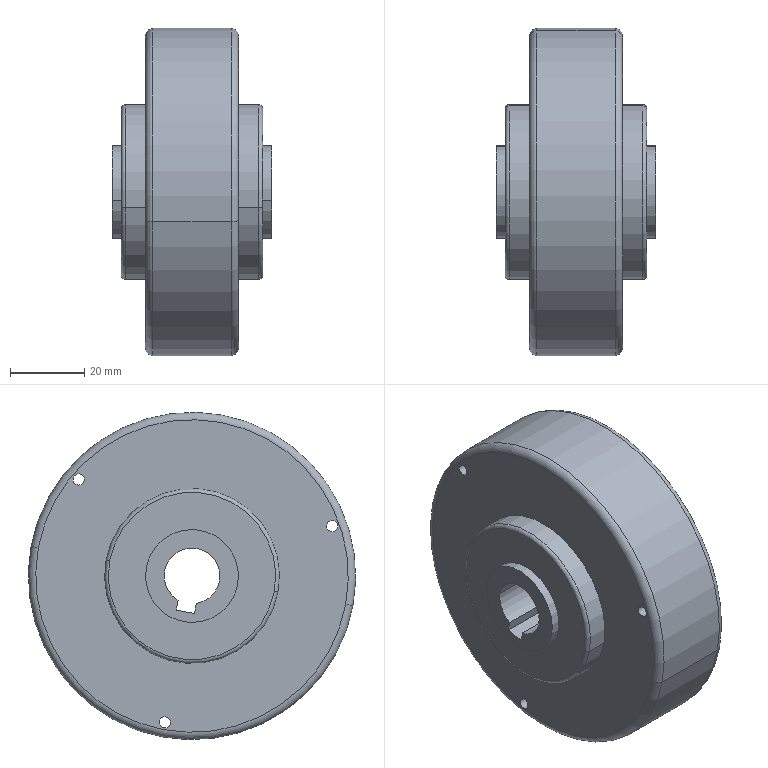Component | SolidWorks | PBT-003-1 | 1 solid | 36 faces | box 43 x 88 x 88 mm | volume 167875 mm3 | cylinder 19 | plane 9 | torus 8 | commonest cylinder face diameters 3 x6 25 x4 47 x4 15 x3 88 x2
build123d program:
from build123d import *

# Parameters (mm, degrees)
SKETCH1_R           = 44
BOSS_EXTRUDE1_DEPTH = 12.5
FILLET1_R           = 2
SKETCH2_R           = 23.5
BOSS_EXTRUDE2_DEPTH = 6.5
FILLET2_R           = 1
BOSS_EXTRUDE3_START = 6.5
SKETCH3_R           = 23.5
BOSS_EXTRUDE3_DEPTH = 6.5
FILLET3_R           = 1
CUT_EXTRUDE1_DEPTH  = 73.911
SKETCH5_R           = 1.5
CUT_EXTRUDE2_DEPTH  = 70.744
BOSS_EXTRUDE5_START = 2.5
SKETCH8_R           = 12.5
BOSS_EXTRUDE5_DEPTH = 2.5


with BuildPart() as part:
    # Sketch1 → Boss-Extrude1 (new, symmetric)
    with BuildSketch(Plane.XY):
        Circle(SKETCH1_R)
    extrude(amount=BOSS_EXTRUDE1_DEPTH, both=True)

    # Fillet1
    fillet1_edges = [part.edges().sort_by_distance(p)[0] for p in [
        (-44, 0, -12.5),
        (-44, 0, 12.5),
    ]]
    fillet(fillet1_edges, radius=FILLET1_R)

    # Sketch2 → Boss-Extrude2 (add)
    with BuildSketch(Plane.XY.offset(12.5)):
        with Locations(Location((0, 0, 0), (0, 0, 180))):
            Circle(SKETCH2_R)
    extrude(amount=BOSS_EXTRUDE2_DEPTH)

    # Fillet2
    fillet2_edges = [part.edges().sort_by_distance(p)[0] for p in [
        (23.5, 0, 19),
    ]]
    fillet(fillet2_edges, radius=FILLET2_R)

    # Sketch3 → Boss-Extrude3 (add)
    with BuildSketch(Plane(origin=(0, 0, -12.5), x_dir=(-1, 0, 0), z_dir=(0, 0, -1)).offset(BOSS_EXTRUDE3_START)):
        Circle(SKETCH3_R)
    extrude(amount=-BOSS_EXTRUDE3_DEPTH)

    # Fillet3
    fillet3_edges = [part.edges().sort_by_distance(p)[0] for p in [
        (23.5, 0, -19),
    ]]
    fillet(fillet3_edges, radius=FILLET3_R)

    # Sketch4 → Cut-Extrude1 (cut, through all)
    with BuildSketch(Plane.XY.offset(19)):
        with BuildLine():
            Line((2.5, 7.071), (2.5, 9.8))
            Line((2.5, 9.8), (-2.5, 9.8))
            Line((-2.5, 9.8), (-2.5, 7.071))
            ThreePointArc((-2.5, 7.071), (0, -7.5), (2.5, 7.071))
        make_face()
    extrude(amount=-CUT_EXTRUDE1_DEPTH, mode=Mode.SUBTRACT)

    # Sketch5 → Cut-Extrude2 (cut, through all)
    with BuildSketch(Plane.XY.offset(12.5)):
        with Locations((0, 40)):
            Circle(SKETCH5_R)
        with Locations((34.641, -20)):
            Circle(SKETCH5_R)
        with Locations((-34.641, -20)):
            Circle(SKETCH5_R)
    extrude(amount=-CUT_EXTRUDE2_DEPTH, mode=Mode.SUBTRACT)

    # Sketch8 → Boss-Extrude5 (add)
    with BuildSketch(Plane.XY.offset(19).offset(BOSS_EXTRUDE5_START)):
        Circle(SKETCH8_R)
        with BuildLine():
            Line((2.5, 7.071), (2.5, 9.8))
            Line((2.5, 9.8), (-2.5, 9.8))
            Line((-2.5, 9.8), (-2.5, 7.071))
            ThreePointArc((-2.5, 7.071), (0, -7.5), (2.5, 7.071))
        make_face(mode=Mode.SUBTRACT)
    boss_extrude5 = extrude(amount=-BOSS_EXTRUDE5_DEPTH)

    # Mirror1: Boss-Extrude5 across plane
    add(boss_extrude5.mirror(Plane.XY))


solid = part.part

# Placed as in the assembly
solid = solid.moved(Location((-51.784, -95.825, 207.018), (-79.544, 90, 0)))
STEP:
#1=CARTESIAN_POINT('',(-1.192,-3.289,8.24));
#2=VERTEX_POINT('',#1);
#3=CARTESIAN_POINT('',(-1.192,-4.257,8.061));
#4=VERTEX_POINT('',#3);
#5=CARTESIAN_POINT('',(-1.192,-3.773,8.15));
#6=DIRECTION('',(-1.,-0.,0.));
#7=DIRECTION('',(-0.,0.9834,0.1815));
#8=AXIS2_PLACEMENT_3D('',#5,#6,#7);
#9=CIRCLE('',#8,0.4921);
#10=EDGE_CURVE('',#2,#4,#9,.T.);
#11=ORIENTED_EDGE('',*,*,#10,.T.);
#12=CARTESIAN_POINT('',(-1.291,-4.257,8.061));
#13=VERTEX_POINT('',#12);
#14=CARTESIAN_POINT('',(-1.192,-4.257,8.061));
#15=DIRECTION('',(-1.,-0.,0.));
#16=VECTOR('',#15,39.37);
#17=LINE('',#14,#16);
#18=EDGE_CURVE('',#4,#13,#17,.T.);
#19=ORIENTED_EDGE('',*,*,#18,.T.);
#20=CARTESIAN_POINT('',(-1.291,-3.289,8.24));
#21=VERTEX_POINT('',#20);
#22=CARTESIAN_POINT('',(-1.291,-3.773,8.15));
#23=DIRECTION('',(1.,0.,-0.));
#24=DIRECTION('',(0.,-0.9834,-0.1815));
#25=AXIS2_PLACEMENT_3D('',#22,#23,#24);
#26=CIRCLE('',#25,0.4921);
#27=EDGE_CURVE('',#13,#21,#26,.T.);
#28=ORIENTED_EDGE('',*,*,#27,.T.);
#29=CARTESIAN_POINT('',(-1.192,-3.289,8.24));
#30=DIRECTION('',(-1.,-0.,0.));
#31=VECTOR('',#30,39.37);
#32=LINE('',#29,#31);
#33=EDGE_CURVE('',#2,#21,#32,.T.);
#34=ORIENTED_EDGE('',*,*,#33,.F.);
#35=EDGE_LOOP('',(#11,#19,#28,#34));
#36=FACE_OUTER_BOUND('',#35,.T.);
#37=CARTESIAN_POINT('',(-1.192,-3.773,8.15));
#38=DIRECTION('',(-1.,-0.,0.));
#39=DIRECTION('',(-0.,0.9834,0.1815));
#40=AXIS2_PLACEMENT_3D('',#37,#38,#39);
#41=CYLINDRICAL_SURFACE('',#40,0.4921);
#42=ADVANCED_FACE('',(#36),#41,.T.);
#43=CARTESIAN_POINT('',(-2.885,-3.289,8.24));
#44=VERTEX_POINT('',#43);
#45=CARTESIAN_POINT('',(-2.885,-4.257,8.061));
#46=VERTEX_POINT('',#45);
#47=CARTESIAN_POINT('',(-2.885,-3.773,8.15));
#48=DIRECTION('',(-1.,-0.,0.));
#49=DIRECTION('',(0.,0.9834,0.1815));
#50=AXIS2_PLACEMENT_3D('',#47,#48,#49);
#51=CIRCLE('',#50,0.4921);
#52=EDGE_CURVE('',#44,#46,#51,.T.);
#53=ORIENTED_EDGE('',*,*,#52,.F.);
#54=CARTESIAN_POINT('',(-2.787,-3.289,8.24));
#55=VERTEX_POINT('',#54);
#56=CARTESIAN_POINT('',(-2.885,-3.289,8.24));
#57=DIRECTION('',(1.,0.,-0.));
#58=VECTOR('',#57,39.37);
#59=LINE('',#56,#58);
#60=EDGE_CURVE('',#44,#55,#59,.T.);
#61=ORIENTED_EDGE('',*,*,#60,.T.);
#62=CARTESIAN_POINT('',(-2.787,-4.257,8.061));
#63=VERTEX_POINT('',#62);
#64=CARTESIAN_POINT('',(-2.787,-3.773,8.15));
#65=DIRECTION('',(-1.,-0.,0.));
#66=DIRECTION('',(0.,0.9834,0.1815));
#67=AXIS2_PLACEMENT_3D('',#64,#65,#66);
#68=CIRCLE('',#67,0.4921);
#69=EDGE_CURVE('',#55,#63,#68,.T.);
#70=ORIENTED_EDGE('',*,*,#69,.T.);
#71=CARTESIAN_POINT('',(-2.885,-4.257,8.061));
#72=DIRECTION('',(1.,0.,-0.));
#73=VECTOR('',#72,39.37);
#74=LINE('',#71,#73);
#75=EDGE_CURVE('',#46,#63,#74,.T.);
#76=ORIENTED_EDGE('',*,*,#75,.F.);
#77=EDGE_LOOP('',(#53,#61,#70,#76));
#78=FACE_OUTER_BOUND('',#77,.T.);
#79=CARTESIAN_POINT('',(-2.885,-3.773,8.15));
#80=DIRECTION('',(1.,0.,-0.));
#81=DIRECTION('',(0.,-0.9834,-0.1815));
#82=AXIS2_PLACEMENT_3D('',#79,#80,#81);
#83=CYLINDRICAL_SURFACE('',#82,0.4921);
#84=ADVANCED_FACE('',(#78),#83,.T.);
#85=CARTESIAN_POINT('',(-1.547,-5.315,8.666));
#86=VERTEX_POINT('',#85);
#87=CARTESIAN_POINT('',(-1.547,-5.199,8.688));
#88=VERTEX_POINT('',#87);
#89=CARTESIAN_POINT('',(-1.547,-5.257,8.677));
#90=DIRECTION('',(-1.,-0.,0.));
#91=DIRECTION('',(0.,0.9834,0.1815));
#92=AXIS2_PLACEMENT_3D('',#89,#90,#91);
#93=CIRCLE('',#92,0.05906);
#94=EDGE_CURVE('',#86,#88,#93,.T.);
#95=ORIENTED_EDGE('',*,*,#94,.F.);
#96=CARTESIAN_POINT('',(-2.531,-5.315,8.666));
#97=VERTEX_POINT('',#96);
#98=CARTESIAN_POINT('',(-1.291,-5.315,8.666));
#99=DIRECTION('',(-1.,-0.,0.));
#100=VECTOR('',#99,39.37);
#101=LINE('',#98,#100);
#102=EDGE_CURVE('',#86,#97,#101,.T.);
#103=ORIENTED_EDGE('',*,*,#102,.T.);
#104=CARTESIAN_POINT('',(-2.531,-5.199,8.688));
#105=VERTEX_POINT('',#104);
#106=CARTESIAN_POINT('',(-2.531,-5.257,8.677));
#107=DIRECTION('',(-1.,-0.,0.));
#108=DIRECTION('',(0.,0.9834,0.1815));
#109=AXIS2_PLACEMENT_3D('',#106,#107,#108);
#110=CIRCLE('',#109,0.05906);
#111=EDGE_CURVE('',#97,#105,#110,.T.);
#112=ORIENTED_EDGE('',*,*,#111,.T.);
#113=CARTESIAN_POINT('',(-1.291,-5.199,8.688));
#114=DIRECTION('',(-1.,-0.,0.));
#115=VECTOR('',#114,39.37);
#116=LINE('',#113,#115);
#117=EDGE_CURVE('',#88,#105,#116,.T.);
#118=ORIENTED_EDGE('',*,*,#117,.F.);
#119=EDGE_LOOP('',(#95,#103,#112,#118));
#120=FACE_OUTER_BOUND('',#119,.T.);
#121=CARTESIAN_POINT('',(-1.291,-5.257,8.677));
#122=DIRECTION('',(-1.,-0.,0.));
#123=DIRECTION('',(0.,0.9834,0.1815));
#124=AXIS2_PLACEMENT_3D('',#121,#122,#123);
#125=CYLINDRICAL_SURFACE('',#124,0.05906);
#126=ADVANCED_FACE('',(#120),#125,.F.);
#127=CARTESIAN_POINT('',(-1.547,-2.632,9.161));
#128=VERTEX_POINT('',#127);
#129=CARTESIAN_POINT('',(-1.547,-2.516,9.183));
#130=VERTEX_POINT('',#129);
#131=CARTESIAN_POINT('',(-1.547,-2.574,9.172));
#132=DIRECTION('',(-1.,-0.,0.));
#133=DIRECTION('',(0.,0.9834,0.1815));
#134=AXIS2_PLACEMENT_3D('',#131,#132,#133);
#135=CIRCLE('',#134,0.05906);
#136=EDGE_CURVE('',#128,#130,#135,.T.);
#137=ORIENTED_EDGE('',*,*,#136,.F.);
#138=CARTESIAN_POINT('',(-2.531,-2.632,9.161));
#139=VERTEX_POINT('',#138);
#140=CARTESIAN_POINT('',(-1.291,-2.632,9.161));
#141=DIRECTION('',(-1.,-0.,0.));
#142=VECTOR('',#141,39.37);
#143=LINE('',#140,#142);
#144=EDGE_CURVE('',#128,#139,#143,.T.);
#145=ORIENTED_EDGE('',*,*,#144,.T.);
#146=CARTESIAN_POINT('',(-2.531,-2.516,9.183));
#147=VERTEX_POINT('',#146);
#148=CARTESIAN_POINT('',(-2.531,-2.574,9.172));
#149=DIRECTION('',(-1.,-0.,0.));
#150=DIRECTION('',(0.,0.9834,0.1815));
#151=AXIS2_PLACEMENT_3D('',#148,#149,#150);
#152=CIRCLE('',#151,0.05906);
#153=EDGE_CURVE('',#139,#147,#152,.T.);
#154=ORIENTED_EDGE('',*,*,#153,.T.);
#155=CARTESIAN_POINT('',(-1.291,-2.516,9.183));
#156=DIRECTION('',(-1.,-0.,0.));
#157=VECTOR('',#156,39.37);
#158=LINE('',#155,#157);
#159=EDGE_CURVE('',#130,#147,#158,.T.);
#160=ORIENTED_EDGE('',*,*,#159,.F.);
#161=EDGE_LOOP('',(#137,#145,#154,#160));
#162=FACE_OUTER_BOUND('',#161,.T.);
#163=CARTESIAN_POINT('',(-1.291,-2.574,9.172));
#164=DIRECTION('',(-1.,-0.,0.));
#165=DIRECTION('',(0.,0.9834,0.1815));
#166=AXIS2_PLACEMENT_3D('',#163,#164,#165);
#167=CYLINDRICAL_SURFACE('',#166,0.05906);
#168=ADVANCED_FACE('',(#162),#167,.F.);
#169=CARTESIAN_POINT('',(-1.547,-3.545,6.591));
#170=VERTEX_POINT('',#169);
#171=CARTESIAN_POINT('',(-1.547,-3.429,6.612));
#172=VERTEX_POINT('',#171);
#173=CARTESIAN_POINT('',(-1.547,-3.487,6.602));
#174=DIRECTION('',(-1.,-0.,0.));
#175=DIRECTION('',(0.,0.9834,0.1815));
#176=AXIS2_PLACEMENT_3D('',#173,#174,#175);
#177=CIRCLE('',#176,0.05906);
#178=EDGE_CURVE('',#170,#172,#177,.T.);
#179=ORIENTED_EDGE('',*,*,#178,.F.);
#180=CARTESIAN_POINT('',(-2.531,-3.545,6.591));
#181=VERTEX_POINT('',#180);
#182=CARTESIAN_POINT('',(-1.291,-3.545,6.591));
#183=DIRECTION('',(-1.,-0.,0.));
#184=VECTOR('',#183,39.37);
#185=LINE('',#182,#184);
#186=EDGE_CURVE('',#170,#181,#185,.T.);
#187=ORIENTED_EDGE('',*,*,#186,.T.);
#188=CARTESIAN_POINT('',(-2.531,-3.429,6.612));
#189=VERTEX_POINT('',#188);
#190=CARTESIAN_POINT('',(-2.531,-3.487,6.602));
#191=DIRECTION('',(-1.,-0.,0.));
#192=DIRECTION('',(0.,0.9834,0.1815));
#193=AXIS2_PLACEMENT_3D('',#190,#191,#192);
#194=CIRCLE('',#193,0.05906);
#195=EDGE_CURVE('',#181,#189,#194,.T.);
#196=ORIENTED_EDGE('',*,*,#195,.T.);
#197=CARTESIAN_POINT('',(-1.291,-3.429,6.612));
#198=DIRECTION('',(-1.,-0.,0.));
#199=VECTOR('',#198,39.37);
#200=LINE('',#197,#199);
#201=EDGE_CURVE('',#172,#189,#200,.T.);
#202=ORIENTED_EDGE('',*,*,#201,.F.);
#203=EDGE_LOOP('',(#179,#187,#196,#202));
#204=FACE_OUTER_BOUND('',#203,.T.);
#205=CARTESIAN_POINT('',(-1.291,-3.487,6.602));
#206=DIRECTION('',(-1.,-0.,0.));
#207=DIRECTION('',(0.,0.9834,0.1815));
#208=AXIS2_PLACEMENT_3D('',#205,#206,#207);
#209=CYLINDRICAL_SURFACE('',#208,0.05906);
#210=ADVANCED_FACE('',(#204),#209,.F.);
#211=CARTESIAN_POINT('',(-1.192,-4.063,8.097));
#212=VERTEX_POINT('',#211);
#213=CARTESIAN_POINT('',(-1.192,-3.482,8.204));
#214=VERTEX_POINT('',#213);
#215=CARTESIAN_POINT('',(-1.192,-3.773,8.15));
#216=DIRECTION('',(-1.,-0.,0.));
#217=DIRECTION('',(-0.,0.9834,0.1815));
#218=AXIS2_PLACEMENT_3D('',#215,#216,#217);
#219=CIRCLE('',#218,0.2953);
#220=EDGE_CURVE('',#212,#214,#219,.T.);
#221=ORIENTED_EDGE('',*,*,#220,.F.);
#222=CARTESIAN_POINT('',(-2.885,-4.063,8.097));
#223=VERTEX_POINT('',#222);
#224=CARTESIAN_POINT('',(-1.291,-4.063,8.097));
#225=DIRECTION('',(-1.,-0.,0.));
#226=VECTOR('',#225,39.37);
#227=LINE('',#224,#226);
#228=EDGE_CURVE('',#212,#223,#227,.T.);
#229=ORIENTED_EDGE('',*,*,#228,.T.);
#230=CARTESIAN_POINT('',(-2.885,-3.482,8.204));
#231=VERTEX_POINT('',#230);
#232=CARTESIAN_POINT('',(-2.885,-3.773,8.15));
#233=DIRECTION('',(-1.,-0.,0.));
#234=DIRECTION('',(0.,0.9834,0.1815));
#235=AXIS2_PLACEMENT_3D('',#232,#233,#234);
#236=CIRCLE('',#235,0.2953);
#237=EDGE_CURVE('',#223,#231,#236,.T.);
#238=ORIENTED_EDGE('',*,*,#237,.T.);
#239=CARTESIAN_POINT('',(-1.291,-3.482,8.204));
#240=DIRECTION('',(-1.,-0.,0.));
#241=VECTOR('',#240,39.37);
#242=LINE('',#239,#241);
#243=EDGE_CURVE('',#214,#231,#242,.T.);
#244=ORIENTED_EDGE('',*,*,#243,.F.);
#245=EDGE_LOOP('',(#221,#229,#238,#244));
#246=FACE_OUTER_BOUND('',#245,.T.);
#247=CARTESIAN_POINT('',(-1.291,-3.773,8.15));
#248=DIRECTION('',(-1.,-0.,0.));
#249=DIRECTION('',(0.,0.9834,0.1815));
#250=AXIS2_PLACEMENT_3D('',#247,#248,#249);
#251=CYLINDRICAL_SURFACE('',#250,0.2953);
#252=ADVANCED_FACE('',(#246),#251,.F.);
#253=CARTESIAN_POINT('',(-1.192,-3.625,7.894));
#254=VERTEX_POINT('',#253);
#255=CARTESIAN_POINT('',(-1.192,-3.773,8.15));
#256=DIRECTION('',(-1.,-0.,0.));
#257=DIRECTION('',(-0.,0.9834,0.1815));
#258=AXIS2_PLACEMENT_3D('',#255,#256,#257);
#259=CIRCLE('',#258,0.2953);
#260=EDGE_CURVE('',#214,#254,#259,.T.);
#261=ORIENTED_EDGE('',*,*,#260,.F.);
#262=ORIENTED_EDGE('',*,*,#243,.T.);
#263=CARTESIAN_POINT('',(-2.885,-3.625,7.894));
#264=VERTEX_POINT('',#263);
#265=CARTESIAN_POINT('',(-2.885,-3.773,8.15));
#266=DIRECTION('',(-1.,-0.,0.));
#267=DIRECTION('',(0.,0.9834,0.1815));
#268=AXIS2_PLACEMENT_3D('',#265,#266,#267);
#269=CIRCLE('',#268,0.2953);
#270=EDGE_CURVE('',#231,#264,#269,.T.);
#271=ORIENTED_EDGE('',*,*,#270,.T.);
#272=CARTESIAN_POINT('',(-1.291,-3.625,7.894));
#273=DIRECTION('',(-1.,-0.,0.));
#274=VECTOR('',#273,39.37);
#275=LINE('',#272,#274);
#276=EDGE_CURVE('',#254,#264,#275,.T.);
#277=ORIENTED_EDGE('',*,*,#276,.F.);
#278=EDGE_LOOP('',(#261,#262,#271,#277));
#279=FACE_OUTER_BOUND('',#278,.T.);
#280=CARTESIAN_POINT('',(-1.291,-3.773,8.15));
#281=DIRECTION('',(-1.,-0.,0.));
#282=DIRECTION('',(0.,0.9834,0.1815));
#283=AXIS2_PLACEMENT_3D('',#280,#281,#282);
#284=CYLINDRICAL_SURFACE('',#283,0.2953);
#285=ADVANCED_FACE('',(#279),#284,.F.);
#286=CARTESIAN_POINT('',(-1.33,-2.863,8.318));
#287=VERTEX_POINT('',#286);
#288=CARTESIAN_POINT('',(-1.33,-4.682,7.982));
#289=VERTEX_POINT('',#288);
#290=CARTESIAN_POINT('',(-1.33,-3.773,8.15));
#291=DIRECTION('',(-1.,-0.,0.));
#292=DIRECTION('',(0.,-0.9834,-0.1815));
#293=AXIS2_PLACEMENT_3D('',#290,#291,#292);
#294=CIRCLE('',#293,0.9252);
#295=EDGE_CURVE('',#287,#289,#294,.T.);
#296=ORIENTED_EDGE('',*,*,#295,.F.);
#297=CARTESIAN_POINT('',(-1.291,-2.902,8.311));
#298=VERTEX_POINT('',#297);
#299=CARTESIAN_POINT('',(-1.33,-2.902,8.311));
#300=DIRECTION('',(-0.,0.1815,-0.9834));
#301=DIRECTION('',(0.,0.9834,0.1815));
#302=AXIS2_PLACEMENT_3D('',#299,#300,#301);
#303=CIRCLE('',#302,0.03937);
#304=EDGE_CURVE('',#287,#298,#303,.T.);
#305=ORIENTED_EDGE('',*,*,#304,.T.);
#306=CARTESIAN_POINT('',(-1.291,-4.644,7.99));
#307=VERTEX_POINT('',#306);
#308=CARTESIAN_POINT('',(-1.291,-3.773,8.15));
#309=DIRECTION('',(1.,0.,-0.));
#310=DIRECTION('',(0.,-0.9834,-0.1815));
#311=AXIS2_PLACEMENT_3D('',#308,#309,#310);
#312=CIRCLE('',#311,0.8858);
#313=EDGE_CURVE('',#307,#298,#312,.T.);
#314=ORIENTED_EDGE('',*,*,#313,.F.);
#315=CARTESIAN_POINT('',(-1.33,-4.644,7.99));
#316=DIRECTION('',(0.,-0.1815,0.9834));
#317=DIRECTION('',(0.,-0.9834,-0.1815));
#318=AXIS2_PLACEMENT_3D('',#315,#316,#317);
#319=CIRCLE('',#318,0.03937);
#320=EDGE_CURVE('',#289,#307,#319,.T.);
#321=ORIENTED_EDGE('',*,*,#320,.F.);
#322=EDGE_LOOP('',(#296,#305,#314,#321));
#323=FACE_OUTER_BOUND('',#322,.T.);
#324=CARTESIAN_POINT('',(-1.33,-3.773,8.15));
#325=DIRECTION('',(1.,0.,-0.));
#326=DIRECTION('',(0.,-0.9834,-0.1815));
#327=AXIS2_PLACEMENT_3D('',#324,#325,#326);
#328=TOROIDAL_SURFACE('',#327,0.8858,0.03937);
#329=ADVANCED_FACE('',(#323),#328,.T.);
#330=ORIENTED_EDGE('',*,*,#295,.T.);
#331=CARTESIAN_POINT('',(-1.547,-4.682,7.982));
#332=VERTEX_POINT('',#331);
#333=CARTESIAN_POINT('',(-1.291,-4.682,7.982));
#334=DIRECTION('',(-1.,-0.,0.));
#335=VECTOR('',#334,39.37);
#336=LINE('',#333,#335);
#337=EDGE_CURVE('',#289,#332,#336,.T.);
#338=ORIENTED_EDGE('',*,*,#337,.T.);
#339=CARTESIAN_POINT('',(-1.547,-2.863,8.318));
#340=VERTEX_POINT('',#339);
#341=CARTESIAN_POINT('',(-1.547,-3.773,8.15));
#342=DIRECTION('',(1.,0.,-0.));
#343=DIRECTION('',(-0.,0.9834,0.1815));
#344=AXIS2_PLACEMENT_3D('',#341,#342,#343);
#345=CIRCLE('',#344,0.9252);
#346=EDGE_CURVE('',#332,#340,#345,.T.);
#347=ORIENTED_EDGE('',*,*,#346,.T.);
#348=CARTESIAN_POINT('',(-1.291,-2.863,8.318));
#349=DIRECTION('',(-1.,-0.,0.));
#350=VECTOR('',#349,39.37);
#351=LINE('',#348,#350);
#352=EDGE_CURVE('',#287,#340,#351,.T.);
#353=ORIENTED_EDGE('',*,*,#352,.F.);
#354=EDGE_LOOP('',(#330,#338,#347,#353));
#355=FACE_OUTER_BOUND('',#354,.T.);
#356=CARTESIAN_POINT('',(-1.291,-3.773,8.15));
#357=DIRECTION('',(-1.,-0.,0.));
#358=DIRECTION('',(-0.,0.9834,0.1815));
#359=AXIS2_PLACEMENT_3D('',#356,#357,#358);
#360=CYLINDRICAL_SURFACE('',#359,0.9252);
#361=ADVANCED_FACE('',(#355),#360,.T.);
#362=CARTESIAN_POINT('',(-2.747,-4.682,7.982));
#363=VERTEX_POINT('',#362);
#364=CARTESIAN_POINT('',(-2.747,-2.863,8.318));
#365=VERTEX_POINT('',#364);
#366=CARTESIAN_POINT('',(-2.747,-3.773,8.15));
#367=DIRECTION('',(1.,0.,-0.));
#368=DIRECTION('',(0.,0.9834,0.1815));
#369=AXIS2_PLACEMENT_3D('',#366,#367,#368);
#370=CIRCLE('',#369,0.9252);
#371=EDGE_CURVE('',#363,#365,#370,.T.);
#372=ORIENTED_EDGE('',*,*,#371,.F.);
#373=CARTESIAN_POINT('',(-2.787,-4.644,7.99));
#374=VERTEX_POINT('',#373);
#375=CARTESIAN_POINT('',(-2.747,-4.644,7.99));
#376=DIRECTION('',(-0.,0.1815,-0.9834));
#377=DIRECTION('',(0.,0.9834,0.1815));
#378=AXIS2_PLACEMENT_3D('',#375,#376,#377);
#379=CIRCLE('',#378,0.03937);
#380=EDGE_CURVE('',#363,#374,#379,.T.);
#381=ORIENTED_EDGE('',*,*,#380,.T.);
#382=CARTESIAN_POINT('',(-2.787,-2.902,8.311));
#383=VERTEX_POINT('',#382);
#384=CARTESIAN_POINT('',(-2.787,-3.773,8.15));
#385=DIRECTION('',(-1.,-0.,0.));
#386=DIRECTION('',(0.,0.9834,0.1815));
#387=AXIS2_PLACEMENT_3D('',#384,#385,#386);
#388=CIRCLE('',#387,0.8858);
#389=EDGE_CURVE('',#383,#374,#388,.T.);
#390=ORIENTED_EDGE('',*,*,#389,.F.);
#391=CARTESIAN_POINT('',(-2.747,-2.902,8.311));
#392=DIRECTION('',(0.,-0.1815,0.9834));
#393=DIRECTION('',(0.,-0.9834,-0.1815));
#394=AXIS2_PLACEMENT_3D('',#391,#392,#393);
#395=CIRCLE('',#394,0.03937);
#396=EDGE_CURVE('',#365,#383,#395,.T.);
#397=ORIENTED_EDGE('',*,*,#396,.F.);
#398=EDGE_LOOP('',(#372,#381,#390,#397));
#399=FACE_OUTER_BOUND('',#398,.T.);
#400=CARTESIAN_POINT('',(-2.747,-3.773,8.15));
#401=DIRECTION('',(-1.,-0.,0.));
#402=DIRECTION('',(-0.,0.9834,0.1815));
#403=AXIS2_PLACEMENT_3D('',#400,#401,#402);
#404=TOROIDAL_SURFACE('',#403,0.8858,0.03937);
#405=ADVANCED_FACE('',(#399),#404,.T.);
#406=ORIENTED_EDGE('',*,*,#371,.T.);
#407=CARTESIAN_POINT('',(-2.531,-2.863,8.318));
#408=VERTEX_POINT('',#407);
#409=CARTESIAN_POINT('',(-2.787,-2.863,8.318));
#410=DIRECTION('',(1.,0.,-0.));
#411=VECTOR('',#410,39.37);
#412=LINE('',#409,#411);
#413=EDGE_CURVE('',#365,#408,#412,.T.);
#414=ORIENTED_EDGE('',*,*,#413,.T.);
#415=CARTESIAN_POINT('',(-2.531,-4.682,7.982));
#416=VERTEX_POINT('',#415);
#417=CARTESIAN_POINT('',(-2.531,-3.773,8.15));
#418=DIRECTION('',(-1.,-0.,0.));
#419=DIRECTION('',(0.,0.9834,0.1815));
#420=AXIS2_PLACEMENT_3D('',#417,#418,#419);
#421=CIRCLE('',#420,0.9252);
#422=EDGE_CURVE('',#408,#416,#421,.T.);
#423=ORIENTED_EDGE('',*,*,#422,.T.);
#424=CARTESIAN_POINT('',(-2.787,-4.682,7.982));
#425=DIRECTION('',(1.,0.,-0.));
#426=VECTOR('',#425,39.37);
#427=LINE('',#424,#426);
#428=EDGE_CURVE('',#363,#416,#427,.T.);
#429=ORIENTED_EDGE('',*,*,#428,.F.);
#430=EDGE_LOOP('',(#406,#414,#423,#429));
#431=FACE_OUTER_BOUND('',#430,.T.);
#432=CARTESIAN_POINT('',(-2.787,-3.773,8.15));
#433=DIRECTION('',(1.,0.,-0.));
#434=DIRECTION('',(0.,-0.9834,-0.1815));
#435=AXIS2_PLACEMENT_3D('',#432,#433,#434);
#436=CYLINDRICAL_SURFACE('',#435,0.9252);
#437=ADVANCED_FACE('',(#431),#436,.T.);
#438=CARTESIAN_POINT('',(-2.452,-5.476,7.836));
#439=VERTEX_POINT('',#438);
#440=CARTESIAN_POINT('',(-2.452,-2.069,8.465));
#441=VERTEX_POINT('',#440);
#442=CARTESIAN_POINT('',(-2.452,-3.773,8.15));
#443=DIRECTION('',(1.,0.,-0.));
#444=DIRECTION('',(-0.,0.9834,0.1815));
#445=AXIS2_PLACEMENT_3D('',#442,#443,#444);
#446=CIRCLE('',#445,1.732);
#447=EDGE_CURVE('',#439,#441,#446,.T.);
#448=ORIENTED_EDGE('',*,*,#447,.F.);
#449=CARTESIAN_POINT('',(-2.531,-5.399,7.85));
#450=VERTEX_POINT('',#449);
#451=CARTESIAN_POINT('',(-2.452,-5.399,7.85));
#452=DIRECTION('',(-0.,0.1815,-0.9834));
#453=DIRECTION('',(0.,0.9834,0.1815));
#454=AXIS2_PLACEMENT_3D('',#451,#452,#453);
#455=CIRCLE('',#454,0.07874);
#456=EDGE_CURVE('',#439,#450,#455,.T.);
#457=ORIENTED_EDGE('',*,*,#456,.T.);
#458=CARTESIAN_POINT('',(-2.531,-2.147,8.45));
#459=VERTEX_POINT('',#458);
#460=CARTESIAN_POINT('',(-2.531,-3.773,8.15));
#461=DIRECTION('',(-1.,-0.,0.));
#462=DIRECTION('',(-0.,0.9834,0.1815));
#463=AXIS2_PLACEMENT_3D('',#460,#461,#462);
#464=CIRCLE('',#463,1.654);
#465=EDGE_CURVE('',#459,#450,#464,.T.);
#466=ORIENTED_EDGE('',*,*,#465,.F.);
#467=CARTESIAN_POINT('',(-2.452,-2.147,8.45));
#468=DIRECTION('',(0.,-0.1815,0.9834));
#469=DIRECTION('',(0.,-0.9834,-0.1815));
#470=AXIS2_PLACEMENT_3D('',#467,#468,#469);
#471=CIRCLE('',#470,0.07874);
#472=EDGE_CURVE('',#441,#459,#471,.T.);
#473=ORIENTED_EDGE('',*,*,#472,.F.);
#474=EDGE_LOOP('',(#448,#457,#466,#473));
#475=FACE_OUTER_BOUND('',#474,.T.);
#476=CARTESIAN_POINT('',(-2.452,-3.773,8.15));
#477=DIRECTION('',(-1.,-0.,0.));
#478=DIRECTION('',(-0.,0.9834,0.1815));
#479=AXIS2_PLACEMENT_3D('',#476,#477,#478);
#480=TOROIDAL_SURFACE('',#479,1.654,0.07874);
#481=ADVANCED_FACE('',(#475),#480,.T.);
#482=CARTESIAN_POINT('',(-1.547,-5.399,7.85));
#483=VERTEX_POINT('',#482);
#484=CARTESIAN_POINT('',(-1.547,-2.147,8.45));
#485=VERTEX_POINT('',#484);
#486=CARTESIAN_POINT('',(-1.547,-3.773,8.15));
#487=DIRECTION('',(1.,0.,-0.));
#488=DIRECTION('',(-0.,0.9834,0.1815));
#489=AXIS2_PLACEMENT_3D('',#486,#487,#488);
#490=CIRCLE('',#489,1.654);
#491=EDGE_CURVE('',#483,#485,#490,.T.);
#492=ORIENTED_EDGE('',*,*,#491,.F.);
#493=CARTESIAN_POINT('',(-1.625,-5.476,7.836));
#494=VERTEX_POINT('',#493);
#495=CARTESIAN_POINT('',(-1.625,-5.399,7.85));
#496=DIRECTION('',(-0.,0.1815,-0.9834));
#497=DIRECTION('',(0.,0.9834,0.1815));
#498=AXIS2_PLACEMENT_3D('',#495,#496,#497);
#499=CIRCLE('',#498,0.07874);
#500=EDGE_CURVE('',#483,#494,#499,.T.);
#501=ORIENTED_EDGE('',*,*,#500,.T.);
#502=CARTESIAN_POINT('',(-1.625,-2.069,8.465));
#503=VERTEX_POINT('',#502);
#504=CARTESIAN_POINT('',(-1.625,-3.773,8.15));
#505=DIRECTION('',(-1.,-0.,0.));
#506=DIRECTION('',(-0.,0.9834,0.1815));
#507=AXIS2_PLACEMENT_3D('',#504,#505,#506);
#508=CIRCLE('',#507,1.732);
#509=EDGE_CURVE('',#503,#494,#508,.T.);
#510=ORIENTED_EDGE('',*,*,#509,.F.);
#511=CARTESIAN_POINT('',(-1.625,-2.147,8.45));
#512=DIRECTION('',(0.,-0.1815,0.9834));
#513=DIRECTION('',(0.,-0.9834,-0.1815));
#514=AXIS2_PLACEMENT_3D('',#511,#512,#513);
#515=CIRCLE('',#514,0.07874);
#516=EDGE_CURVE('',#485,#503,#515,.T.);
#517=ORIENTED_EDGE('',*,*,#516,.F.);
#518=EDGE_LOOP('',(#492,#501,#510,#517));
#519=FACE_OUTER_BOUND('',#518,.T.);
#520=CARTESIAN_POINT('',(-1.625,-3.773,8.15));
#521=DIRECTION('',(-1.,-0.,0.));
#522=DIRECTION('',(-0.,0.9834,0.1815));
#523=AXIS2_PLACEMENT_3D('',#520,#521,#522);
#524=TOROIDAL_SURFACE('',#523,1.654,0.07874);
#525=ADVANCED_FACE('',(#519),#524,.T.);
#526=ORIENTED_EDGE('',*,*,#447,.T.);
#527=CARTESIAN_POINT('',(-2.531,-2.069,8.465));
#528=DIRECTION('',(1.,0.,-0.));
#529=VECTOR('',#528,39.37);
#530=LINE('',#527,#529);
#531=EDGE_CURVE('',#441,#503,#530,.T.);
#532=ORIENTED_EDGE('',*,*,#531,.T.);
#533=ORIENTED_EDGE('',*,*,#509,.T.);
#534=CARTESIAN_POINT('',(-2.531,-5.476,7.836));
#535=DIRECTION('',(1.,0.,-0.));
#536=VECTOR('',#535,39.37);
#537=LINE('',#534,#536);
#538=EDGE_CURVE('',#439,#494,#537,.T.);
#539=ORIENTED_EDGE('',*,*,#538,.F.);
#540=EDGE_LOOP('',(#526,#532,#533,#539));
#541=FACE_OUTER_BOUND('',#540,.T.);
#542=CARTESIAN_POINT('',(-2.531,-3.773,8.15));
#543=DIRECTION('',(1.,0.,-0.));
#544=DIRECTION('',(0.,-0.9834,-0.1815));
#545=AXIS2_PLACEMENT_3D('',#542,#543,#544);
#546=CYLINDRICAL_SURFACE('',#545,1.732);
#547=ADVANCED_FACE('',(#541),#546,.T.);
#548=ORIENTED_EDGE('',*,*,#389,.T.);
#549=CARTESIAN_POINT('',(-2.787,-3.773,8.15));
#550=DIRECTION('',(-1.,-0.,0.));
#551=DIRECTION('',(0.,0.9834,0.1815));
#552=AXIS2_PLACEMENT_3D('',#549,#550,#551);
#553=CIRCLE('',#552,0.8858);
#554=EDGE_CURVE('',#374,#383,#553,.T.);
#555=ORIENTED_EDGE('',*,*,#554,.T.);
#556=EDGE_LOOP('',(#548,#555));
#557=FACE_OUTER_BOUND('',#556,.T.);
#558=CARTESIAN_POINT('',(-2.787,-3.773,8.15));
#559=DIRECTION('',(-1.,-0.,0.));
#560=DIRECTION('',(0.,0.9834,0.1815));
#561=AXIS2_PLACEMENT_3D('',#558,#559,#560);
#562=CIRCLE('',#561,0.4921);
#563=EDGE_CURVE('',#63,#55,#562,.T.);
#564=ORIENTED_EDGE('',*,*,#563,.F.);
#565=ORIENTED_EDGE('',*,*,#69,.F.);
#566=EDGE_LOOP('',(#564,#565));
#567=FACE_BOUND('',#566,.T.);
#568=CARTESIAN_POINT('',(-2.787,-3.773,8.15));
#569=DIRECTION('',(-1.,-0.,0.));
#570=DIRECTION('',(-0.,0.9834,0.1815));
#571=AXIS2_PLACEMENT_3D('',#568,#569,#570);
#572=PLANE('',#571);
#573=ADVANCED_FACE('',(#557,#567),#572,.T.);
#574=CARTESIAN_POINT('',(-1.547,-5.257,8.677));
#575=DIRECTION('',(-1.,-0.,0.));
#576=DIRECTION('',(0.,0.9834,0.1815));
#577=AXIS2_PLACEMENT_3D('',#574,#575,#576);
#578=CIRCLE('',#577,0.05906);
#579=EDGE_CURVE('',#88,#86,#578,.T.);
#580=ORIENTED_EDGE('',*,*,#579,.T.);
#581=ORIENTED_EDGE('',*,*,#94,.T.);
#582=EDGE_LOOP('',(#580,#581));
#583=FACE_BOUND('',#582,.T.);
#584=CARTESIAN_POINT('',(-1.547,-2.574,9.172));
#585=DIRECTION('',(-1.,-0.,0.));
#586=DIRECTION('',(0.,0.9834,0.1815));
#587=AXIS2_PLACEMENT_3D('',#584,#585,#586);
#588=CIRCLE('',#587,0.05906);
#589=EDGE_CURVE('',#130,#128,#588,.T.);
#590=ORIENTED_EDGE('',*,*,#589,.T.);
#591=ORIENTED_EDGE('',*,*,#136,.T.);
#592=EDGE_LOOP('',(#590,#591));
#593=FACE_BOUND('',#592,.T.);
#594=CARTESIAN_POINT('',(-1.547,-3.487,6.602));
#595=DIRECTION('',(-1.,-0.,0.));
#596=DIRECTION('',(0.,0.9834,0.1815));
#597=AXIS2_PLACEMENT_3D('',#594,#595,#596);
#598=CIRCLE('',#597,0.05906);
#599=EDGE_CURVE('',#172,#170,#598,.T.);
#600=ORIENTED_EDGE('',*,*,#599,.T.);
#601=ORIENTED_EDGE('',*,*,#178,.T.);
#602=EDGE_LOOP('',(#600,#601));
#603=FACE_BOUND('',#602,.T.);
#604=CARTESIAN_POINT('',(-1.547,-3.773,8.15));
#605=DIRECTION('',(1.,0.,-0.));
#606=DIRECTION('',(-0.,0.9834,0.1815));
#607=AXIS2_PLACEMENT_3D('',#604,#605,#606);
#608=CIRCLE('',#607,1.654);
#609=EDGE_CURVE('',#485,#483,#608,.T.);
#610=ORIENTED_EDGE('',*,*,#609,.T.);
#611=ORIENTED_EDGE('',*,*,#491,.T.);
#612=EDGE_LOOP('',(#610,#611));
#613=FACE_OUTER_BOUND('',#612,.T.);
#614=CARTESIAN_POINT('',(-1.547,-3.773,8.15));
#615=DIRECTION('',(1.,0.,-0.));
#616=DIRECTION('',(-0.,0.9834,0.1815));
#617=AXIS2_PLACEMENT_3D('',#614,#615,#616);
#618=CIRCLE('',#617,0.9252);
#619=EDGE_CURVE('',#340,#332,#618,.T.);
#620=ORIENTED_EDGE('',*,*,#619,.F.);
#621=ORIENTED_EDGE('',*,*,#346,.F.);
#622=EDGE_LOOP('',(#620,#621));
#623=FACE_BOUND('',#622,.T.);
#624=CARTESIAN_POINT('',(-1.547,-3.773,8.15));
#625=DIRECTION('',(-1.,-0.,0.));
#626=DIRECTION('',(-0.,0.9834,0.1815));
#627=AXIS2_PLACEMENT_3D('',#624,#625,#626);
#628=PLANE('',#627);
#629=ADVANCED_FACE('',(#583,#593,#603,#613,#623),#628,.F.);
#630=CARTESIAN_POINT('',(-2.531,-5.257,8.677));
#631=DIRECTION('',(-1.,-0.,0.));
#632=DIRECTION('',(0.,0.9834,0.1815));
#633=AXIS2_PLACEMENT_3D('',#630,#631,#632);
#634=CIRCLE('',#633,0.05906);
#635=EDGE_CURVE('',#105,#97,#634,.T.);
#636=ORIENTED_EDGE('',*,*,#635,.F.);
#637=ORIENTED_EDGE('',*,*,#111,.F.);
#638=EDGE_LOOP('',(#636,#637));
#639=FACE_BOUND('',#638,.T.);
#640=CARTESIAN_POINT('',(-2.531,-2.574,9.172));
#641=DIRECTION('',(-1.,-0.,0.));
#642=DIRECTION('',(0.,0.9834,0.1815));
#643=AXIS2_PLACEMENT_3D('',#640,#641,#642);
#644=CIRCLE('',#643,0.05906);
#645=EDGE_CURVE('',#147,#139,#644,.T.);
#646=ORIENTED_EDGE('',*,*,#645,.F.);
#647=ORIENTED_EDGE('',*,*,#153,.F.);
#648=EDGE_LOOP('',(#646,#647));
#649=FACE_BOUND('',#648,.T.);
#650=CARTESIAN_POINT('',(-2.531,-3.487,6.602));
#651=DIRECTION('',(-1.,-0.,0.));
#652=DIRECTION('',(0.,0.9834,0.1815));
#653=AXIS2_PLACEMENT_3D('',#650,#651,#652);
#654=CIRCLE('',#653,0.05906);
#655=EDGE_CURVE('',#189,#181,#654,.T.);
#656=ORIENTED_EDGE('',*,*,#655,.F.);
#657=ORIENTED_EDGE('',*,*,#195,.F.);
#658=EDGE_LOOP('',(#656,#657));
#659=FACE_BOUND('',#658,.T.);
#660=ORIENTED_EDGE('',*,*,#465,.T.);
#661=CARTESIAN_POINT('',(-2.531,-3.773,8.15));
#662=DIRECTION('',(-1.,-0.,0.));
#663=DIRECTION('',(-0.,0.9834,0.1815));
#664=AXIS2_PLACEMENT_3D('',#661,#662,#663);
#665=CIRCLE('',#664,1.654);
#666=EDGE_CURVE('',#450,#459,#665,.T.);
#667=ORIENTED_EDGE('',*,*,#666,.T.);
#668=EDGE_LOOP('',(#660,#667));
#669=FACE_OUTER_BOUND('',#668,.T.);
#670=CARTESIAN_POINT('',(-2.531,-3.773,8.15));
#671=DIRECTION('',(-1.,-0.,0.));
#672=DIRECTION('',(0.,0.9834,0.1815));
#673=AXIS2_PLACEMENT_3D('',#670,#671,#672);
#674=CIRCLE('',#673,0.9252);
#675=EDGE_CURVE('',#416,#408,#674,.T.);
#676=ORIENTED_EDGE('',*,*,#675,.F.);
#677=ORIENTED_EDGE('',*,*,#422,.F.);
#678=EDGE_LOOP('',(#676,#677));
#679=FACE_BOUND('',#678,.T.);
#680=CARTESIAN_POINT('',(-2.531,-3.773,8.15));
#681=DIRECTION('',(-1.,-0.,0.));
#682=DIRECTION('',(-0.,0.9834,0.1815));
#683=AXIS2_PLACEMENT_3D('',#680,#681,#682);
#684=PLANE('',#683);
#685=ADVANCED_FACE('',(#639,#649,#659,#669,#679),#684,.T.);
#686=ORIENTED_EDGE('',*,*,#531,.F.);
#687=CARTESIAN_POINT('',(-2.452,-3.773,8.15));
#688=DIRECTION('',(1.,0.,-0.));
#689=DIRECTION('',(-0.,0.9834,0.1815));
#690=AXIS2_PLACEMENT_3D('',#687,#688,#689);
#691=CIRCLE('',#690,1.732);
#692=EDGE_CURVE('',#441,#439,#691,.T.);
#693=ORIENTED_EDGE('',*,*,#692,.T.);
#694=ORIENTED_EDGE('',*,*,#538,.T.);
#695=CARTESIAN_POINT('',(-1.625,-3.773,8.15));
#696=DIRECTION('',(-1.,-0.,0.));
#697=DIRECTION('',(-0.,0.9834,0.1815));
#698=AXIS2_PLACEMENT_3D('',#695,#696,#697);
#699=CIRCLE('',#698,1.732);
#700=EDGE_CURVE('',#494,#503,#699,.T.);
#701=ORIENTED_EDGE('',*,*,#700,.T.);
#702=EDGE_LOOP('',(#686,#693,#694,#701));
#703=FACE_OUTER_BOUND('',#702,.T.);
#704=CARTESIAN_POINT('',(-2.531,-3.773,8.15));
#705=DIRECTION('',(1.,0.,-0.));
#706=DIRECTION('',(0.,-0.9834,-0.1815));
#707=AXIS2_PLACEMENT_3D('',#704,#705,#706);
#708=CYLINDRICAL_SURFACE('',#707,1.732);
#709=ADVANCED_FACE('',(#703),#708,.T.);
#710=ORIENTED_EDGE('',*,*,#500,.F.);
#711=ORIENTED_EDGE('',*,*,#609,.F.);
#712=ORIENTED_EDGE('',*,*,#516,.T.);
#713=ORIENTED_EDGE('',*,*,#700,.F.);
#714=EDGE_LOOP('',(#710,#711,#712,#713));
#715=FACE_OUTER_BOUND('',#714,.T.);
#716=CARTESIAN_POINT('',(-1.625,-3.773,8.15));
#717=DIRECTION('',(-1.,-0.,0.));
#718=DIRECTION('',(-0.,0.9834,0.1815));
#719=AXIS2_PLACEMENT_3D('',#716,#717,#718);
#720=TOROIDAL_SURFACE('',#719,1.654,0.07874);
#721=ADVANCED_FACE('',(#715),#720,.T.);
#722=ORIENTED_EDGE('',*,*,#456,.F.);
#723=ORIENTED_EDGE('',*,*,#692,.F.);
#724=ORIENTED_EDGE('',*,*,#472,.T.);
#725=ORIENTED_EDGE('',*,*,#666,.F.);
#726=EDGE_LOOP('',(#722,#723,#724,#725));
#727=FACE_OUTER_BOUND('',#726,.T.);
#728=CARTESIAN_POINT('',(-2.452,-3.773,8.15));
#729=DIRECTION('',(-1.,-0.,0.));
#730=DIRECTION('',(-0.,0.9834,0.1815));
#731=AXIS2_PLACEMENT_3D('',#728,#729,#730);
#732=TOROIDAL_SURFACE('',#731,1.654,0.07874);
#733=ADVANCED_FACE('',(#727),#732,.T.);
#734=ORIENTED_EDGE('',*,*,#413,.F.);
#735=CARTESIAN_POINT('',(-2.747,-3.773,8.15));
#736=DIRECTION('',(1.,0.,-0.));
#737=DIRECTION('',(0.,0.9834,0.1815));
#738=AXIS2_PLACEMENT_3D('',#735,#736,#737);
#739=CIRCLE('',#738,0.9252);
#740=EDGE_CURVE('',#365,#363,#739,.T.);
#741=ORIENTED_EDGE('',*,*,#740,.T.);
#742=ORIENTED_EDGE('',*,*,#428,.T.);
#743=ORIENTED_EDGE('',*,*,#675,.T.);
#744=EDGE_LOOP('',(#734,#741,#742,#743));
#745=FACE_OUTER_BOUND('',#744,.T.);
#746=CARTESIAN_POINT('',(-2.787,-3.773,8.15));
#747=DIRECTION('',(1.,0.,-0.));
#748=DIRECTION('',(0.,-0.9834,-0.1815));
#749=AXIS2_PLACEMENT_3D('',#746,#747,#748);
#750=CYLINDRICAL_SURFACE('',#749,0.9252);
#751=ADVANCED_FACE('',(#745),#750,.T.);
#752=ORIENTED_EDGE('',*,*,#380,.F.);
#753=ORIENTED_EDGE('',*,*,#740,.F.);
#754=ORIENTED_EDGE('',*,*,#396,.T.);
#755=ORIENTED_EDGE('',*,*,#554,.F.);
#756=EDGE_LOOP('',(#752,#753,#754,#755));
#757=FACE_OUTER_BOUND('',#756,.T.);
#758=CARTESIAN_POINT('',(-2.747,-3.773,8.15));
#759=DIRECTION('',(-1.,-0.,0.));
#760=DIRECTION('',(-0.,0.9834,0.1815));
#761=AXIS2_PLACEMENT_3D('',#758,#759,#760);
#762=TOROIDAL_SURFACE('',#761,0.8858,0.03937);
#763=ADVANCED_FACE('',(#757),#762,.T.);
#764=ORIENTED_EDGE('',*,*,#337,.F.);
#765=CARTESIAN_POINT('',(-1.33,-3.773,8.15));
#766=DIRECTION('',(-1.,-0.,0.));
#767=DIRECTION('',(0.,-0.9834,-0.1815));
#768=AXIS2_PLACEMENT_3D('',#765,#766,#767);
#769=CIRCLE('',#768,0.9252);
#770=EDGE_CURVE('',#289,#287,#769,.T.);
#771=ORIENTED_EDGE('',*,*,#770,.T.);
#772=ORIENTED_EDGE('',*,*,#352,.T.);
#773=ORIENTED_EDGE('',*,*,#619,.T.);
#774=EDGE_LOOP('',(#764,#771,#772,#773));
#775=FACE_OUTER_BOUND('',#774,.T.);
#776=CARTESIAN_POINT('',(-1.291,-3.773,8.15));
#777=DIRECTION('',(-1.,-0.,0.));
#778=DIRECTION('',(-0.,0.9834,0.1815));
#779=AXIS2_PLACEMENT_3D('',#776,#777,#778);
#780=CYLINDRICAL_SURFACE('',#779,0.9252);
#781=ADVANCED_FACE('',(#775),#780,.T.);
#782=CARTESIAN_POINT('',(-1.291,-3.773,8.15));
#783=DIRECTION('',(1.,0.,-0.));
#784=DIRECTION('',(0.,-0.9834,-0.1815));
#785=AXIS2_PLACEMENT_3D('',#782,#783,#784);
#786=CIRCLE('',#785,0.4921);
#787=EDGE_CURVE('',#21,#13,#786,.T.);
#788=ORIENTED_EDGE('',*,*,#787,.F.);
#789=ORIENTED_EDGE('',*,*,#27,.F.);
#790=EDGE_LOOP('',(#788,#789));
#791=FACE_BOUND('',#790,.T.);
#792=ORIENTED_EDGE('',*,*,#313,.T.);
#793=CARTESIAN_POINT('',(-1.291,-3.773,8.15));
#794=DIRECTION('',(1.,0.,-0.));
#795=DIRECTION('',(0.,-0.9834,-0.1815));
#796=AXIS2_PLACEMENT_3D('',#793,#794,#795);
#797=CIRCLE('',#796,0.8858);
#798=EDGE_CURVE('',#298,#307,#797,.T.);
#799=ORIENTED_EDGE('',*,*,#798,.T.);
#800=EDGE_LOOP('',(#792,#799));
#801=FACE_OUTER_BOUND('',#800,.T.);
#802=CARTESIAN_POINT('',(-1.291,-3.773,8.15));
#803=DIRECTION('',(1.,0.,-0.));
#804=DIRECTION('',(0.,-0.9834,-0.1815));
#805=AXIS2_PLACEMENT_3D('',#802,#803,#804);
#806=PLANE('',#805);
#807=ADVANCED_FACE('',(#791,#801),#806,.T.);
#808=ORIENTED_EDGE('',*,*,#304,.F.);
#809=ORIENTED_EDGE('',*,*,#770,.F.);
#810=ORIENTED_EDGE('',*,*,#320,.T.);
#811=ORIENTED_EDGE('',*,*,#798,.F.);
#812=EDGE_LOOP('',(#808,#809,#810,#811));
#813=FACE_OUTER_BOUND('',#812,.T.);
#814=CARTESIAN_POINT('',(-1.33,-3.773,8.15));
#815=DIRECTION('',(1.,0.,-0.));
#816=DIRECTION('',(0.,-0.9834,-0.1815));
#817=AXIS2_PLACEMENT_3D('',#814,#815,#816);
#818=TOROIDAL_SURFACE('',#817,0.8858,0.03937);
#819=ADVANCED_FACE('',(#813),#818,.T.);
#820=ORIENTED_EDGE('',*,*,#228,.F.);
#821=CARTESIAN_POINT('',(-1.192,-3.819,7.859));
#822=VERTEX_POINT('',#821);
#823=CARTESIAN_POINT('',(-1.192,-3.773,8.15));
#824=DIRECTION('',(-1.,-0.,0.));
#825=DIRECTION('',(-0.,0.9834,0.1815));
#826=AXIS2_PLACEMENT_3D('',#823,#824,#825);
#827=CIRCLE('',#826,0.2953);
#828=EDGE_CURVE('',#822,#212,#827,.T.);
#829=ORIENTED_EDGE('',*,*,#828,.F.);
#830=CARTESIAN_POINT('',(-2.885,-3.819,7.859));
#831=VERTEX_POINT('',#830);
#832=CARTESIAN_POINT('',(-1.291,-3.819,7.859));
#833=DIRECTION('',(-1.,-0.,0.));
#834=VECTOR('',#833,39.37);
#835=LINE('',#832,#834);
#836=EDGE_CURVE('',#822,#831,#835,.T.);
#837=ORIENTED_EDGE('',*,*,#836,.T.);
#838=CARTESIAN_POINT('',(-2.885,-3.773,8.15));
#839=DIRECTION('',(-1.,-0.,0.));
#840=DIRECTION('',(0.,0.9834,0.1815));
#841=AXIS2_PLACEMENT_3D('',#838,#839,#840);
#842=CIRCLE('',#841,0.2953);
#843=EDGE_CURVE('',#831,#223,#842,.T.);
#844=ORIENTED_EDGE('',*,*,#843,.T.);
#845=EDGE_LOOP('',(#820,#829,#837,#844));
#846=FACE_OUTER_BOUND('',#845,.T.);
#847=CARTESIAN_POINT('',(-1.291,-3.773,8.15));
#848=DIRECTION('',(-1.,-0.,0.));
#849=DIRECTION('',(0.,0.9834,0.1815));
#850=AXIS2_PLACEMENT_3D('',#847,#848,#849);
#851=CYLINDRICAL_SURFACE('',#850,0.2953);
#852=ADVANCED_FACE('',(#846),#851,.F.);
#853=CARTESIAN_POINT('',(-1.192,-3.799,7.753));
#854=VERTEX_POINT('',#853);
#855=CARTESIAN_POINT('',(-2.885,-3.799,7.753));
#856=VERTEX_POINT('',#855);
#857=CARTESIAN_POINT('',(-1.291,-3.799,7.753));
#858=DIRECTION('',(-1.,-0.,0.));
#859=VECTOR('',#858,39.37);
#860=LINE('',#857,#859);
#861=EDGE_CURVE('',#854,#856,#860,.T.);
#862=ORIENTED_EDGE('',*,*,#861,.T.);
#863=CARTESIAN_POINT('',(-2.885,-3.799,7.753));
#864=DIRECTION('',(0.,-0.1815,0.9834));
#865=VECTOR('',#864,39.37);
#866=LINE('',#863,#865);
#867=EDGE_CURVE('',#856,#831,#866,.T.);
#868=ORIENTED_EDGE('',*,*,#867,.T.);
#869=ORIENTED_EDGE('',*,*,#836,.F.);
#870=CARTESIAN_POINT('',(-1.192,-3.799,7.753));
#871=DIRECTION('',(0.,-0.1815,0.9834));
#872=VECTOR('',#871,39.37);
#873=LINE('',#870,#872);
#874=EDGE_CURVE('',#854,#822,#873,.T.);
#875=ORIENTED_EDGE('',*,*,#874,.F.);
#876=EDGE_LOOP('',(#862,#868,#869,#875));
#877=FACE_OUTER_BOUND('',#876,.T.);
#878=CARTESIAN_POINT('',(-1.291,-3.819,7.859));
#879=DIRECTION('',(0.,-0.9834,-0.1815));
#880=DIRECTION('',(-1.,-0.,0.));
#881=AXIS2_PLACEMENT_3D('',#878,#879,#880);
#882=PLANE('',#881);
#883=ADVANCED_FACE('',(#877),#882,.F.);
#884=CARTESIAN_POINT('',(-1.192,-3.606,7.789));
#885=VERTEX_POINT('',#884);
#886=CARTESIAN_POINT('',(-2.885,-3.606,7.789));
#887=VERTEX_POINT('',#886);
#888=CARTESIAN_POINT('',(-1.291,-3.606,7.789));
#889=DIRECTION('',(-1.,-0.,0.));
#890=VECTOR('',#889,39.37);
#891=LINE('',#888,#890);
#892=EDGE_CURVE('',#885,#887,#891,.T.);
#893=ORIENTED_EDGE('',*,*,#892,.T.);
#894=CARTESIAN_POINT('',(-2.885,-3.606,7.789));
#895=DIRECTION('',(0.,-0.9834,-0.1815));
#896=VECTOR('',#895,39.37);
#897=LINE('',#894,#896);
#898=EDGE_CURVE('',#887,#856,#897,.T.);
#899=ORIENTED_EDGE('',*,*,#898,.T.);
#900=ORIENTED_EDGE('',*,*,#861,.F.);
#901=CARTESIAN_POINT('',(-1.192,-3.606,7.789));
#902=DIRECTION('',(0.,-0.9834,-0.1815));
#903=VECTOR('',#902,39.37);
#904=LINE('',#901,#903);
#905=EDGE_CURVE('',#885,#854,#904,.T.);
#906=ORIENTED_EDGE('',*,*,#905,.F.);
#907=EDGE_LOOP('',(#893,#899,#900,#906));
#908=FACE_OUTER_BOUND('',#907,.T.);
#909=CARTESIAN_POINT('',(-1.291,-3.799,7.753));
#910=DIRECTION('',(-0.,0.1815,-0.9834));
#911=DIRECTION('',(-1.,-0.,0.));
#912=AXIS2_PLACEMENT_3D('',#909,#910,#911);
#913=PLANE('',#912);
#914=ADVANCED_FACE('',(#908),#913,.F.);
#915=ORIENTED_EDGE('',*,*,#276,.T.);
#916=CARTESIAN_POINT('',(-2.885,-3.625,7.894));
#917=DIRECTION('',(-0.,0.1815,-0.9834));
#918=VECTOR('',#917,39.37);
#919=LINE('',#916,#918);
#920=EDGE_CURVE('',#264,#887,#919,.T.);
#921=ORIENTED_EDGE('',*,*,#920,.T.);
#922=ORIENTED_EDGE('',*,*,#892,.F.);
#923=CARTESIAN_POINT('',(-1.192,-3.625,7.894));
#924=DIRECTION('',(-0.,0.1815,-0.9834));
#925=VECTOR('',#924,39.37);
#926=LINE('',#923,#925);
#927=EDGE_CURVE('',#254,#885,#926,.T.);
#928=ORIENTED_EDGE('',*,*,#927,.F.);
#929=EDGE_LOOP('',(#915,#921,#922,#928));
#930=FACE_OUTER_BOUND('',#929,.T.);
#931=CARTESIAN_POINT('',(-1.291,-3.625,7.894));
#932=DIRECTION('',(-0.,0.9834,0.1815));
#933=DIRECTION('',(1.,0.,-0.));
#934=AXIS2_PLACEMENT_3D('',#931,#932,#933);
#935=PLANE('',#934);
#936=ADVANCED_FACE('',(#930),#935,.F.);
#937=ORIENTED_EDGE('',*,*,#186,.F.);
#938=ORIENTED_EDGE('',*,*,#599,.F.);
#939=ORIENTED_EDGE('',*,*,#201,.T.);
#940=ORIENTED_EDGE('',*,*,#655,.T.);
#941=EDGE_LOOP('',(#937,#938,#939,#940));
#942=FACE_OUTER_BOUND('',#941,.T.);
#943=CARTESIAN_POINT('',(-1.291,-3.487,6.602));
#944=DIRECTION('',(-1.,-0.,0.));
#945=DIRECTION('',(0.,0.9834,0.1815));
#946=AXIS2_PLACEMENT_3D('',#943,#944,#945);
#947=CYLINDRICAL_SURFACE('',#946,0.05906);
#948=ADVANCED_FACE('',(#942),#947,.F.);
#949=ORIENTED_EDGE('',*,*,#144,.F.);
#950=ORIENTED_EDGE('',*,*,#589,.F.);
#951=ORIENTED_EDGE('',*,*,#159,.T.);
#952=ORIENTED_EDGE('',*,*,#645,.T.);
#953=EDGE_LOOP('',(#949,#950,#951,#952));
#954=FACE_OUTER_BOUND('',#953,.T.);
#955=CARTESIAN_POINT('',(-1.291,-2.574,9.172));
#956=DIRECTION('',(-1.,-0.,0.));
#957=DIRECTION('',(0.,0.9834,0.1815));
#958=AXIS2_PLACEMENT_3D('',#955,#956,#957);
#959=CYLINDRICAL_SURFACE('',#958,0.05906);
#960=ADVANCED_FACE('',(#954),#959,.F.);
#961=ORIENTED_EDGE('',*,*,#102,.F.);
#962=ORIENTED_EDGE('',*,*,#579,.F.);
#963=ORIENTED_EDGE('',*,*,#117,.T.);
#964=ORIENTED_EDGE('',*,*,#635,.T.);
#965=EDGE_LOOP('',(#961,#962,#963,#964));
#966=FACE_OUTER_BOUND('',#965,.T.);
#967=CARTESIAN_POINT('',(-1.291,-5.257,8.677));
#968=DIRECTION('',(-1.,-0.,0.));
#969=DIRECTION('',(0.,0.9834,0.1815));
#970=AXIS2_PLACEMENT_3D('',#967,#968,#969);
#971=CYLINDRICAL_SURFACE('',#970,0.05906);
#972=ADVANCED_FACE('',(#966),#971,.F.);
#973=CARTESIAN_POINT('',(-2.885,-3.773,8.15));
#974=DIRECTION('',(-1.,-0.,0.));
#975=DIRECTION('',(0.,0.9834,0.1815));
#976=AXIS2_PLACEMENT_3D('',#973,#974,#975);
#977=CIRCLE('',#976,0.4921);
#978=EDGE_CURVE('',#46,#44,#977,.T.);
#979=ORIENTED_EDGE('',*,*,#978,.T.);
#980=ORIENTED_EDGE('',*,*,#52,.T.);
#981=EDGE_LOOP('',(#979,#980));
#982=FACE_OUTER_BOUND('',#981,.T.);
#983=ORIENTED_EDGE('',*,*,#920,.F.);
#984=ORIENTED_EDGE('',*,*,#270,.F.);
#985=ORIENTED_EDGE('',*,*,#237,.F.);
#986=ORIENTED_EDGE('',*,*,#843,.F.);
#987=ORIENTED_EDGE('',*,*,#867,.F.);
#988=ORIENTED_EDGE('',*,*,#898,.F.);
#989=EDGE_LOOP('',(#983,#984,#985,#986,#987,#988));
#990=FACE_BOUND('',#989,.T.);
#991=CARTESIAN_POINT('',(-2.885,-3.773,8.15));
#992=DIRECTION('',(-1.,-0.,0.));
#993=DIRECTION('',(-0.,0.9834,0.1815));
#994=AXIS2_PLACEMENT_3D('',#991,#992,#993);
#995=PLANE('',#994);
#996=ADVANCED_FACE('',(#982,#990),#995,.T.);
#997=ORIENTED_EDGE('',*,*,#60,.F.);
#998=ORIENTED_EDGE('',*,*,#978,.F.);
#999=ORIENTED_EDGE('',*,*,#75,.T.);
#1000=ORIENTED_EDGE('',*,*,#563,.T.);
#1001=EDGE_LOOP('',(#997,#998,#999,#1000));
#1002=FACE_OUTER_BOUND('',#1001,.T.);
#1003=CARTESIAN_POINT('',(-2.885,-3.773,8.15));
#1004=DIRECTION('',(1.,0.,-0.));
#1005=DIRECTION('',(0.,-0.9834,-0.1815));
#1006=AXIS2_PLACEMENT_3D('',#1003,#1004,#1005);
#1007=CYLINDRICAL_SURFACE('',#1006,0.4921);
#1008=ADVANCED_FACE('',(#1002),#1007,.T.);
#1009=ORIENTED_EDGE('',*,*,#18,.F.);
#1010=CARTESIAN_POINT('',(-1.192,-3.773,8.15));
#1011=DIRECTION('',(-1.,-0.,0.));
#1012=DIRECTION('',(-0.,0.9834,0.1815));
#1013=AXIS2_PLACEMENT_3D('',#1010,#1011,#1012);
#1014=CIRCLE('',#1013,0.4921);
#1015=EDGE_CURVE('',#4,#2,#1014,.T.);
#1016=ORIENTED_EDGE('',*,*,#1015,.T.);
#1017=ORIENTED_EDGE('',*,*,#33,.T.);
#1018=ORIENTED_EDGE('',*,*,#787,.T.);
#1019=EDGE_LOOP('',(#1009,#1016,#1017,#1018));
#1020=FACE_OUTER_BOUND('',#1019,.T.);
#1021=CARTESIAN_POINT('',(-1.192,-3.773,8.15));
#1022=DIRECTION('',(-1.,-0.,0.));
#1023=DIRECTION('',(-0.,0.9834,0.1815));
#1024=AXIS2_PLACEMENT_3D('',#1021,#1022,#1023);
#1025=CYLINDRICAL_SURFACE('',#1024,0.4921);
#1026=ADVANCED_FACE('',(#1020),#1025,.T.);
#1027=ORIENTED_EDGE('',*,*,#828,.T.);
#1028=ORIENTED_EDGE('',*,*,#220,.T.);
#1029=ORIENTED_EDGE('',*,*,#260,.T.);
#1030=ORIENTED_EDGE('',*,*,#927,.T.);
#1031=ORIENTED_EDGE('',*,*,#905,.T.);
#1032=ORIENTED_EDGE('',*,*,#874,.T.);
#1033=EDGE_LOOP('',(#1027,#1028,#1029,#1030,#1031,#1032));
#1034=FACE_BOUND('',#1033,.T.);
#1035=ORIENTED_EDGE('',*,*,#10,.F.);
#1036=ORIENTED_EDGE('',*,*,#1015,.F.);
#1037=EDGE_LOOP('',(#1035,#1036));
#1038=FACE_OUTER_BOUND('',#1037,.T.);
#1039=CARTESIAN_POINT('',(-1.192,-3.773,8.15));
#1040=DIRECTION('',(1.,0.,-0.));
#1041=DIRECTION('',(-0.,0.9834,0.1815));
#1042=AXIS2_PLACEMENT_3D('',#1039,#1040,#1041);
#1043=PLANE('',#1042);
#1044=ADVANCED_FACE('',(#1034,#1038),#1043,.T.);
#1045=CLOSED_SHELL('',(#42,#84,#126,#168,#210,#252,#285,#329,#361,#405,#437,#481,#525,#547,#573,#629,#685,#709,#721,#733,#751,#763,#781,#807,#819,#852,#883,#914,#936,#948,#960,#972,#996,#1008,#1026,#1044));
#1046=MANIFOLD_SOLID_BREP('',#1045);
#1047=CARTESIAN_POINT('',(0.,0.,0.));
#1048=DIRECTION('',(0.,0.,1.));
#1049=DIRECTION('',(1.,0.,0.));
#1050=AXIS2_PLACEMENT_3D('',#1047,#1048,#1049);
#1051=(LENGTH_UNIT()NAMED_UNIT(*)SI_UNIT($,.METRE.));
#1052=LENGTH_MEASURE_WITH_UNIT(LENGTH_MEASURE(0.0254),#1051);
#1053=DIMENSIONAL_EXPONENTS(1.,0.,0.,0.,0.,0.,0.);
#1054=(CONVERSION_BASED_UNIT('',#1052)LENGTH_UNIT()NAMED_UNIT(#1053));
#1055=UNCERTAINTY_MEASURE_WITH_UNIT(LENGTH_MEASURE(0.00001),#1054,'','');
#1056=(NAMED_UNIT(*)PLANE_ANGLE_UNIT()SI_UNIT($,.RADIAN.));
#1057=(NAMED_UNIT(*)SI_UNIT($,.STERADIAN.)SOLID_ANGLE_UNIT());
#1058=(GEOMETRIC_REPRESENTATION_CONTEXT(3)GLOBAL_UNCERTAINTY_ASSIGNED_CONTEXT((#1055))GLOBAL_UNIT_ASSIGNED_CONTEXT((#1054,#1056,#1057))REPRESENTATION_CONTEXT('',''));
#1059=ADVANCED_BREP_SHAPE_REPRESENTATION('',(#1046,#1050),#1058);
#1060=COLOUR_RGB('',0.7922,0.8196,0.9333);
#1061=FILL_AREA_STYLE_COLOUR('',#1060);
#1062=FILL_AREA_STYLE('',(#1061));
#1063=SURFACE_STYLE_FILL_AREA(#1062);
#1064=SURFACE_SIDE_STYLE('',(#1063));
#1065=SURFACE_STYLE_USAGE(.BOTH.,#1064);
#1066=PRESENTATION_STYLE_ASSIGNMENT((#1065));
#1067=STYLED_ITEM('',(#1066),#1046);
#1068=(LENGTH_UNIT()NAMED_UNIT(*)SI_UNIT($,.METRE.));
#1069=LENGTH_MEASURE_WITH_UNIT(LENGTH_MEASURE(0.0254),#1068);
#1070=DIMENSIONAL_EXPONENTS(1.,0.,0.,0.,0.,0.,0.);
#1071=(CONVERSION_BASED_UNIT('',#1069)LENGTH_UNIT()NAMED_UNIT(#1070));
#1072=UNCERTAINTY_MEASURE_WITH_UNIT(LENGTH_MEASURE(0.00001),#1071,'','');
#1073=(NAMED_UNIT(*)PLANE_ANGLE_UNIT()SI_UNIT($,.RADIAN.));
#1074=(NAMED_UNIT(*)SI_UNIT($,.STERADIAN.)SOLID_ANGLE_UNIT());
#1075=(GEOMETRIC_REPRESENTATION_CONTEXT(3)GLOBAL_UNCERTAINTY_ASSIGNED_CONTEXT((#1072))GLOBAL_UNIT_ASSIGNED_CONTEXT((#1071,#1073,#1074))REPRESENTATION_CONTEXT('',''));
#1076=MECHANICAL_DESIGN_GEOMETRIC_PRESENTATION_REPRESENTATION('',(#1067),#1075);
#1077=PRESENTATION_LAYER_ASSIGNMENT('','',(#1067));